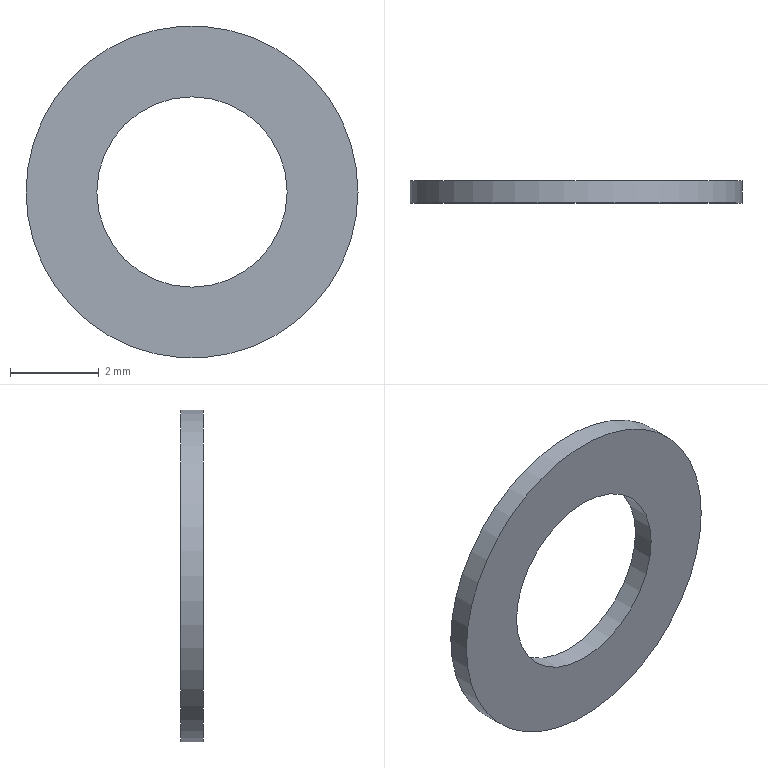Component | NX | SPRING_WASHER_4 | 1 solid | 4 faces | box 7.5 x 0.5 x 7.5 mm | volume 15 mm3 | cylinder 2 | plane 2 | commonest cylinder face diameters 7.5 x1 4.3 x1
STEP:
#1=CARTESIAN_POINT('',(0.,0.,0.));
#2=DIRECTION('',(0.,0.,1.));
#3=DIRECTION('',(1.,0.,0.));
#4=AXIS2_PLACEMENT_3D('',#1,#2,#3);
#5=CARTESIAN_POINT('',(29.75,-31.5,7.5));
#6=VERTEX_POINT('',#5);
#7=CARTESIAN_POINT('',(26.,-31.5,7.5));
#8=DIRECTION('',(0.,1.,0.));
#9=DIRECTION('',(1.,0.,0.));
#10=AXIS2_PLACEMENT_3D('',#7,#8,#9);
#11=CIRCLE('',#10,3.75);
#12=CARTESIAN_POINT('',(26.,-31.5,7.5));
#13=DIRECTION('',(0.,1.,0.));
#14=DIRECTION('',(-1.,0.,0.));
#15=AXIS2_PLACEMENT_3D('',#12,#13,#14);
#16=CYLINDRICAL_SURFACE('',#15,3.75);
#17=CARTESIAN_POINT('',(3.142,0.));
#18=DIRECTION('',(1.,0.));
#19=VECTOR('',#18,1.);
#20=LINE('',#17,#19);
#21=(GEOMETRIC_REPRESENTATION_CONTEXT(2)PARAMETRIC_REPRESENTATION_CONTEXT()REPRESENTATION_CONTEXT('',''));
#22=DEFINITIONAL_REPRESENTATION('',(#20),#21);
#23=PCURVE('',#16,#22);
#24=CARTESIAN_POINT('',(26.,-31.5,7.5));
#25=DIRECTION('',(0.,1.,0.));
#26=DIRECTION('',(-1.,0.,0.));
#27=AXIS2_PLACEMENT_3D('',#24,#25,#26);
#28=PLANE('',#27);
#29=CARTESIAN_POINT('',(0.,0.));
#30=DIRECTION('',(-1.,0.));
#31=AXIS2_PLACEMENT_2D('',#29,#30);
#32=CIRCLE('',#31,3.75);
#33=(GEOMETRIC_REPRESENTATION_CONTEXT(2)PARAMETRIC_REPRESENTATION_CONTEXT()REPRESENTATION_CONTEXT('',''));
#34=DEFINITIONAL_REPRESENTATION('',(#32),#33);
#35=PCURVE('',#28,#34);
#36=SURFACE_CURVE('',#11,(#23,#35),.PCURVE_S1.);
#37=EDGE_CURVE('',#6,#6,#36,.T.);
#38=ORIENTED_EDGE('',*,*,#37,.T.);
#39=CARTESIAN_POINT('',(29.75,-31.,7.5));
#40=VERTEX_POINT('',#39);
#41=CARTESIAN_POINT('',(29.75,-31.5,7.5));
#42=CARTESIAN_POINT('',(29.75,-31.,7.5));
#43=B_SPLINE_CURVE_WITH_KNOTS('',1,(#41,#42),.UNSPECIFIED.,.F.,.F.,(2,2),(0.,0.5),.PIECEWISE_BEZIER_KNOTS.);
#44=CARTESIAN_POINT('',(9.425,0.));
#45=DIRECTION('',(0.,1.));
#46=VECTOR('',#45,1.);
#47=LINE('',#44,#46);
#48=(GEOMETRIC_REPRESENTATION_CONTEXT(2)PARAMETRIC_REPRESENTATION_CONTEXT()REPRESENTATION_CONTEXT('',''));
#49=DEFINITIONAL_REPRESENTATION('',(#47),#48);
#50=PCURVE('',#16,#49);
#51=CARTESIAN_POINT('',(3.142,0.));
#52=DIRECTION('',(0.,1.));
#53=VECTOR('',#52,1.);
#54=LINE('',#51,#53);
#55=(GEOMETRIC_REPRESENTATION_CONTEXT(2)PARAMETRIC_REPRESENTATION_CONTEXT()REPRESENTATION_CONTEXT('',''));
#56=DEFINITIONAL_REPRESENTATION('',(#54),#55);
#57=PCURVE('',#16,#56);
#58=SEAM_CURVE('',#43,(#50,#57),.PCURVE_S1.);
#59=EDGE_CURVE('',#6,#40,#58,.T.);
#60=ORIENTED_EDGE('',*,*,#59,.T.);
#61=CARTESIAN_POINT('',(26.,-31.,7.5));
#62=DIRECTION('',(0.,1.,0.));
#63=DIRECTION('',(1.,0.,0.));
#64=AXIS2_PLACEMENT_3D('',#61,#62,#63);
#65=CIRCLE('',#64,3.75);
#66=CARTESIAN_POINT('',(3.142,0.5));
#67=DIRECTION('',(1.,0.));
#68=VECTOR('',#67,1.);
#69=LINE('',#66,#68);
#70=(GEOMETRIC_REPRESENTATION_CONTEXT(2)PARAMETRIC_REPRESENTATION_CONTEXT()REPRESENTATION_CONTEXT('',''));
#71=DEFINITIONAL_REPRESENTATION('',(#69),#70);
#72=PCURVE('',#16,#71);
#73=CARTESIAN_POINT('',(26.,-31.,7.5));
#74=DIRECTION('',(0.,1.,0.));
#75=DIRECTION('',(-1.,0.,0.));
#76=AXIS2_PLACEMENT_3D('',#73,#74,#75);
#77=PLANE('',#76);
#78=CARTESIAN_POINT('',(0.,0.));
#79=DIRECTION('',(-1.,0.));
#80=AXIS2_PLACEMENT_2D('',#78,#79);
#81=CIRCLE('',#80,3.75);
#82=(GEOMETRIC_REPRESENTATION_CONTEXT(2)PARAMETRIC_REPRESENTATION_CONTEXT()REPRESENTATION_CONTEXT('',''));
#83=DEFINITIONAL_REPRESENTATION('',(#81),#82);
#84=PCURVE('',#77,#83);
#85=SURFACE_CURVE('',#65,(#72,#84),.PCURVE_S1.);
#86=EDGE_CURVE('',#40,#40,#85,.T.);
#87=ORIENTED_EDGE('',*,*,#86,.F.);
#88=ORIENTED_EDGE('',*,*,#59,.F.);
#89=EDGE_LOOP('',(#38,#60,#87,#88));
#90=FACE_BOUND('',#89,.T.);
#91=ADVANCED_FACE('',(#90),#16,.T.);
#92=CARTESIAN_POINT('',(28.15,-31.5,7.5));
#93=VERTEX_POINT('',#92);
#94=CARTESIAN_POINT('',(26.,-31.5,7.5));
#95=DIRECTION('',(0.,1.,0.));
#96=DIRECTION('',(1.,0.,0.));
#97=AXIS2_PLACEMENT_3D('',#94,#95,#96);
#98=CIRCLE('',#97,2.15);
#99=CARTESIAN_POINT('',(26.,-31.5,7.5));
#100=DIRECTION('',(0.,1.,0.));
#101=DIRECTION('',(-1.,0.,0.));
#102=AXIS2_PLACEMENT_3D('',#99,#100,#101);
#103=CYLINDRICAL_SURFACE('',#102,2.15);
#104=CARTESIAN_POINT('',(3.142,0.));
#105=DIRECTION('',(1.,0.));
#106=VECTOR('',#105,1.);
#107=LINE('',#104,#106);
#108=(GEOMETRIC_REPRESENTATION_CONTEXT(2)PARAMETRIC_REPRESENTATION_CONTEXT()REPRESENTATION_CONTEXT('',''));
#109=DEFINITIONAL_REPRESENTATION('',(#107),#108);
#110=PCURVE('',#103,#109);
#111=CARTESIAN_POINT('',(0.,0.));
#112=DIRECTION('',(-1.,0.));
#113=AXIS2_PLACEMENT_2D('',#111,#112);
#114=CIRCLE('',#113,2.15);
#115=(GEOMETRIC_REPRESENTATION_CONTEXT(2)PARAMETRIC_REPRESENTATION_CONTEXT()REPRESENTATION_CONTEXT('',''));
#116=DEFINITIONAL_REPRESENTATION('',(#114),#115);
#117=PCURVE('',#28,#116);
#118=SURFACE_CURVE('',#98,(#110,#117),.PCURVE_S1.);
#119=EDGE_CURVE('',#93,#93,#118,.T.);
#120=ORIENTED_EDGE('',*,*,#119,.T.);
#121=CARTESIAN_POINT('',(28.15,-31.,7.5));
#122=VERTEX_POINT('',#121);
#123=CARTESIAN_POINT('',(28.15,-31.5,7.5));
#124=CARTESIAN_POINT('',(28.15,-31.,7.5));
#125=B_SPLINE_CURVE_WITH_KNOTS('',1,(#123,#124),.UNSPECIFIED.,.F.,.F.,(2,2),(0.,0.5),.PIECEWISE_BEZIER_KNOTS.);
#126=CARTESIAN_POINT('',(9.425,0.));
#127=DIRECTION('',(0.,1.));
#128=VECTOR('',#127,1.);
#129=LINE('',#126,#128);
#130=(GEOMETRIC_REPRESENTATION_CONTEXT(2)PARAMETRIC_REPRESENTATION_CONTEXT()REPRESENTATION_CONTEXT('',''));
#131=DEFINITIONAL_REPRESENTATION('',(#129),#130);
#132=PCURVE('',#103,#131);
#133=CARTESIAN_POINT('',(3.142,0.));
#134=DIRECTION('',(0.,1.));
#135=VECTOR('',#134,1.);
#136=LINE('',#133,#135);
#137=(GEOMETRIC_REPRESENTATION_CONTEXT(2)PARAMETRIC_REPRESENTATION_CONTEXT()REPRESENTATION_CONTEXT('',''));
#138=DEFINITIONAL_REPRESENTATION('',(#136),#137);
#139=PCURVE('',#103,#138);
#140=SEAM_CURVE('',#125,(#132,#139),.PCURVE_S1.);
#141=EDGE_CURVE('',#93,#122,#140,.T.);
#142=ORIENTED_EDGE('',*,*,#141,.T.);
#143=CARTESIAN_POINT('',(26.,-31.,7.5));
#144=DIRECTION('',(0.,1.,0.));
#145=DIRECTION('',(1.,0.,0.));
#146=AXIS2_PLACEMENT_3D('',#143,#144,#145);
#147=CIRCLE('',#146,2.15);
#148=CARTESIAN_POINT('',(3.142,0.5));
#149=DIRECTION('',(1.,0.));
#150=VECTOR('',#149,1.);
#151=LINE('',#148,#150);
#152=(GEOMETRIC_REPRESENTATION_CONTEXT(2)PARAMETRIC_REPRESENTATION_CONTEXT()REPRESENTATION_CONTEXT('',''));
#153=DEFINITIONAL_REPRESENTATION('',(#151),#152);
#154=PCURVE('',#103,#153);
#155=CARTESIAN_POINT('',(0.,0.));
#156=DIRECTION('',(-1.,0.));
#157=AXIS2_PLACEMENT_2D('',#155,#156);
#158=CIRCLE('',#157,2.15);
#159=(GEOMETRIC_REPRESENTATION_CONTEXT(2)PARAMETRIC_REPRESENTATION_CONTEXT()REPRESENTATION_CONTEXT('',''));
#160=DEFINITIONAL_REPRESENTATION('',(#158),#159);
#161=PCURVE('',#77,#160);
#162=SURFACE_CURVE('',#147,(#154,#161),.PCURVE_S1.);
#163=EDGE_CURVE('',#122,#122,#162,.T.);
#164=ORIENTED_EDGE('',*,*,#163,.F.);
#165=ORIENTED_EDGE('',*,*,#141,.F.);
#166=EDGE_LOOP('',(#120,#142,#164,#165));
#167=FACE_BOUND('',#166,.F.);
#168=ADVANCED_FACE('',(#167),#103,.F.);
#169=ORIENTED_EDGE('',*,*,#37,.F.);
#170=EDGE_LOOP('',(#169));
#171=FACE_BOUND('',#170,.T.);
#172=ORIENTED_EDGE('',*,*,#119,.T.);
#173=EDGE_LOOP('',(#172));
#174=FACE_BOUND('',#173,.T.);
#175=ADVANCED_FACE('',(#171,#174),#28,.F.);
#176=ORIENTED_EDGE('',*,*,#86,.T.);
#177=EDGE_LOOP('',(#176));
#178=FACE_BOUND('',#177,.T.);
#179=ORIENTED_EDGE('',*,*,#163,.F.);
#180=EDGE_LOOP('',(#179));
#181=FACE_BOUND('',#180,.T.);
#182=ADVANCED_FACE('',(#178,#181),#77,.T.);
#183=CLOSED_SHELL('',(#91,#168,#175,#182));
#184=MANIFOLD_SOLID_BREP('',#183);
#185=(LENGTH_UNIT()NAMED_UNIT(*)SI_UNIT(.MILLI.,.METRE.));
#186=UNCERTAINTY_MEASURE_WITH_UNIT(LENGTH_MEASURE(0.00001),#185,'','');
#187=(NAMED_UNIT(*)PLANE_ANGLE_UNIT()SI_UNIT($,.RADIAN.));
#188=(NAMED_UNIT(*)SI_UNIT($,.STERADIAN.)SOLID_ANGLE_UNIT());
#189=(GEOMETRIC_REPRESENTATION_CONTEXT(3)GLOBAL_UNCERTAINTY_ASSIGNED_CONTEXT((#186))GLOBAL_UNIT_ASSIGNED_CONTEXT((#185,#187,#188))REPRESENTATION_CONTEXT('',''));
#190=ADVANCED_BREP_SHAPE_REPRESENTATION('',(#4,#184),#189);